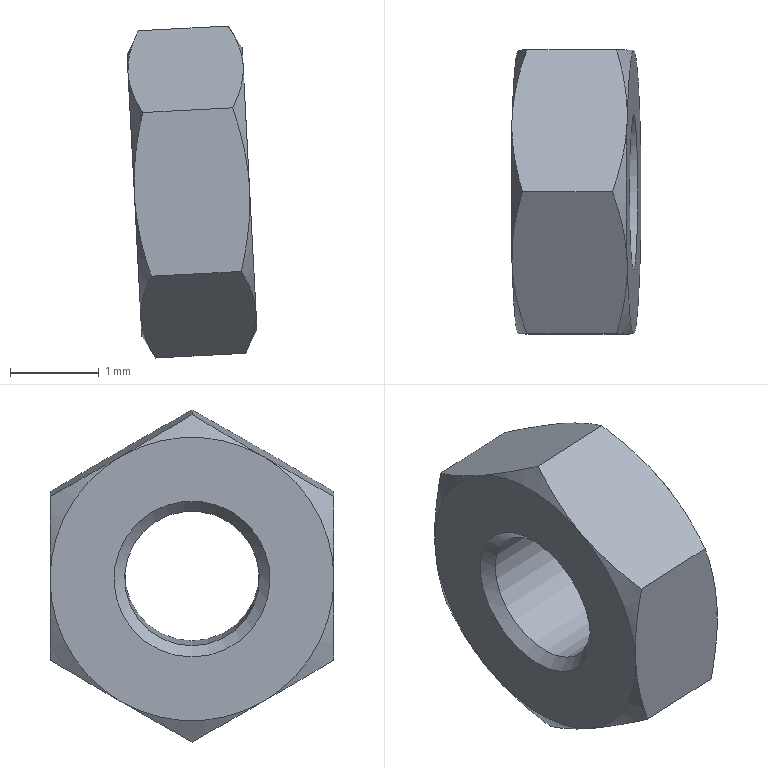Component | NX | GB-T6170_F-2000_M1_6X0_35 | 1 solid | 23 faces | volume 9 mm3 | cone 14 | plane 8 | cylinder 1 | commonest cylinder face diameters 1.52 x1